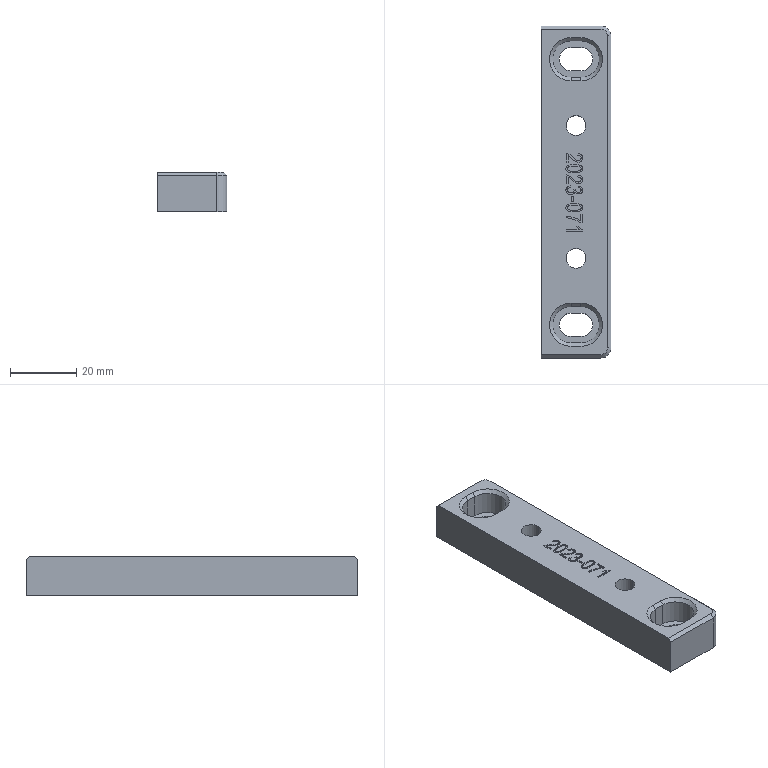CAM job | Mastercam | mm | 14 operations | part box 25 x 106 x 12
1. Facing | 1 - 50 J面铣
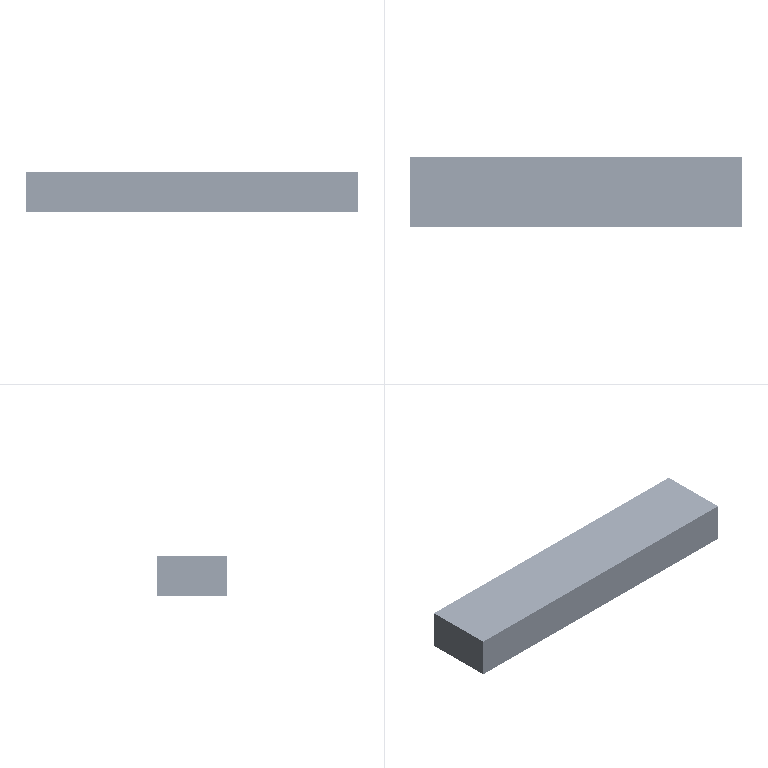2. 2D High Speed (2D Dynamic Mill) | 9 - 10C 平底刀
3. Contour (Ramp) | 6 - 6 平底刀
4. Contour (Ramp) | 7 - 4 平底刀
5. Helix Bore | 7 - 4 平底刀
6. Contour (2D) | 6 - 6 平底刀
7. Contour (2D) | 11 - 4 J平底刀
8. Contour (2D) | 10 - 10J 平底刀
9. Helix Bore | 11 - 4 J平底刀
10. Contour (2D chamfer) | 2 - 6定位倒角
11. Contour (2D chamfer) | 2 - 6定位倒角
12. Model Chamfer | 2 - 6定位倒角
13. Facing | 1 - 50 J面铣
14. Model Chamfer | 2 - 6定位倒角